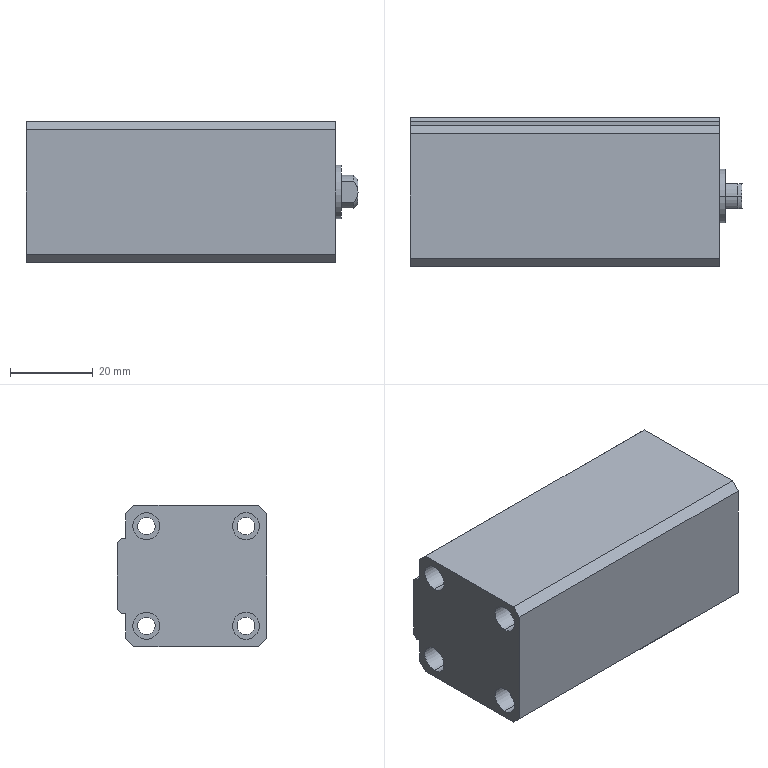Component | SolidWorks | DoubleFilmTransport-1_SDA20X55-2 | 1 solid | 78 faces | volume 83139 mm3 | cylinder 35 | plane 28 | cone 15 | commonest cylinder face diameters 6.5 x16 4.2 x12 8 x3 13 x2 3.3 x2